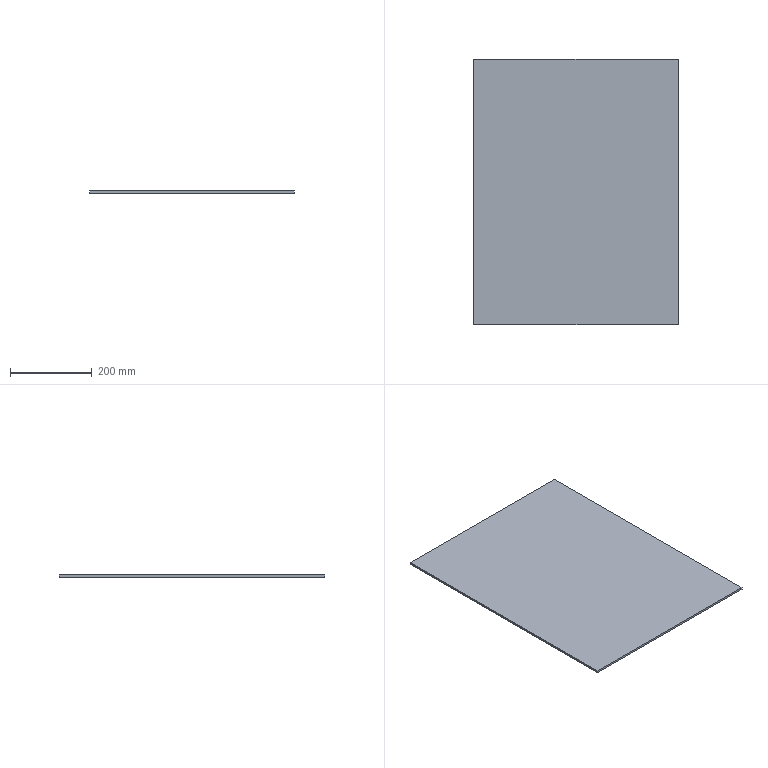Component | SolidWorks | BrownAcrylicPlate-5_BrownAcrylicPlate-5-1 | 1 solid | 6 faces | box 500 x 650 x 5 mm | volume 1625000 mm3 | plane 6
build123d program:
from build123d import *

# Parameters (mm, degrees)
SKETCH1_W           = 500
SKETCH1_H           = 650
BOSS_EXTRUDE1_DEPTH = 5


with BuildPart() as part:
    # Sketch1 → Boss-Extrude1 (new body)
    with BuildSketch(Plane(origin=(0, 0, 0), x_dir=(1, 0, 0), z_dir=(0, 1, 0))):
        Rectangle(SKETCH1_W, SKETCH1_H)
    extrude(amount=BOSS_EXTRUDE1_DEPTH)


solid = part.part

# Placed as in the assembly
solid = solid.moved(Location((335.689, 1675.552, -2328.5), (90, 0, 0)))
STEP:
#1=COLOUR_RGB('',0.7922,0.8196,0.9333);
#2=FILL_AREA_STYLE_COLOUR('',#1);
#3=FILL_AREA_STYLE('',(#2));
#4=SURFACE_STYLE_FILL_AREA(#3);
#5=SURFACE_SIDE_STYLE('',(#4));
#6=SURFACE_STYLE_USAGE(.BOTH.,#5);
#7=PRESENTATION_STYLE_ASSIGNMENT((#6));
#8=CARTESIAN_POINT('',(23.059,53.171,-91.673));
#9=VERTEX_POINT('',#8);
#10=CARTESIAN_POINT('',(23.059,78.762,-91.673));
#11=VERTEX_POINT('',#10);
#12=CARTESIAN_POINT('',(23.059,78.762,-91.673));
#13=DIRECTION('',(0.,1.,-0.));
#14=VECTOR('',#13,39.37);
#15=LINE('',#12,#14);
#16=EDGE_CURVE('',#9,#11,#15,.T.);
#17=ORIENTED_EDGE('',*,*,#16,.T.);
#18=CARTESIAN_POINT('',(23.059,78.762,-91.476));
#19=VERTEX_POINT('',#18);
#20=CARTESIAN_POINT('',(23.059,78.762,-91.476));
#21=DIRECTION('',(-0.,-0.,-1.));
#22=VECTOR('',#21,39.37);
#23=LINE('',#20,#22);
#24=EDGE_CURVE('',#19,#11,#23,.T.);
#25=ORIENTED_EDGE('',*,*,#24,.F.);
#26=CARTESIAN_POINT('',(23.059,53.171,-91.476));
#27=VERTEX_POINT('',#26);
#28=CARTESIAN_POINT('',(23.059,78.762,-91.476));
#29=DIRECTION('',(0.,1.,-0.));
#30=VECTOR('',#29,39.37);
#31=LINE('',#28,#30);
#32=EDGE_CURVE('',#27,#19,#31,.T.);
#33=ORIENTED_EDGE('',*,*,#32,.F.);
#34=CARTESIAN_POINT('',(23.059,53.171,-91.476));
#35=DIRECTION('',(-0.,-0.,-1.));
#36=VECTOR('',#35,39.37);
#37=LINE('',#34,#36);
#38=EDGE_CURVE('',#27,#9,#37,.T.);
#39=ORIENTED_EDGE('',*,*,#38,.T.);
#40=EDGE_LOOP('',(#17,#25,#33,#39));
#41=FACE_OUTER_BOUND('',#40,.T.);
#42=CARTESIAN_POINT('',(23.059,78.762,-91.476));
#43=DIRECTION('',(-1.,0.,0.));
#44=DIRECTION('',(-0.,-1.,0.));
#45=AXIS2_PLACEMENT_3D('',#42,#43,#44);
#46=PLANE('',#45);
#47=ADVANCED_FACE('',(#41),#46,.F.);
#48=CARTESIAN_POINT('',(3.374,78.762,-91.673));
#49=VERTEX_POINT('',#48);
#50=CARTESIAN_POINT('',(3.374,78.762,-91.673));
#51=DIRECTION('',(-1.,0.,0.));
#52=VECTOR('',#51,39.37);
#53=LINE('',#50,#52);
#54=EDGE_CURVE('',#11,#49,#53,.T.);
#55=ORIENTED_EDGE('',*,*,#54,.T.);
#56=CARTESIAN_POINT('',(3.374,78.762,-91.476));
#57=VERTEX_POINT('',#56);
#58=CARTESIAN_POINT('',(3.374,78.762,-91.476));
#59=DIRECTION('',(-0.,-0.,-1.));
#60=VECTOR('',#59,39.37);
#61=LINE('',#58,#60);
#62=EDGE_CURVE('',#57,#49,#61,.T.);
#63=ORIENTED_EDGE('',*,*,#62,.F.);
#64=CARTESIAN_POINT('',(3.374,78.762,-91.476));
#65=DIRECTION('',(-1.,0.,0.));
#66=VECTOR('',#65,39.37);
#67=LINE('',#64,#66);
#68=EDGE_CURVE('',#19,#57,#67,.T.);
#69=ORIENTED_EDGE('',*,*,#68,.F.);
#70=ORIENTED_EDGE('',*,*,#24,.T.);
#71=EDGE_LOOP('',(#55,#63,#69,#70));
#72=FACE_OUTER_BOUND('',#71,.T.);
#73=CARTESIAN_POINT('',(3.374,78.762,-91.476));
#74=DIRECTION('',(-0.,-1.,0.));
#75=DIRECTION('',(1.,-0.,-0.));
#76=AXIS2_PLACEMENT_3D('',#73,#74,#75);
#77=PLANE('',#76);
#78=ADVANCED_FACE('',(#72),#77,.F.);
#79=CARTESIAN_POINT('',(3.374,53.171,-91.673));
#80=VERTEX_POINT('',#79);
#81=CARTESIAN_POINT('',(3.374,78.762,-91.673));
#82=DIRECTION('',(-0.,-1.,0.));
#83=VECTOR('',#82,39.37);
#84=LINE('',#81,#83);
#85=EDGE_CURVE('',#49,#80,#84,.T.);
#86=ORIENTED_EDGE('',*,*,#85,.T.);
#87=CARTESIAN_POINT('',(3.374,53.171,-91.476));
#88=VERTEX_POINT('',#87);
#89=CARTESIAN_POINT('',(3.374,53.171,-91.476));
#90=DIRECTION('',(-0.,-0.,-1.));
#91=VECTOR('',#90,39.37);
#92=LINE('',#89,#91);
#93=EDGE_CURVE('',#88,#80,#92,.T.);
#94=ORIENTED_EDGE('',*,*,#93,.F.);
#95=CARTESIAN_POINT('',(3.374,78.762,-91.476));
#96=DIRECTION('',(-0.,-1.,0.));
#97=VECTOR('',#96,39.37);
#98=LINE('',#95,#97);
#99=EDGE_CURVE('',#57,#88,#98,.T.);
#100=ORIENTED_EDGE('',*,*,#99,.F.);
#101=ORIENTED_EDGE('',*,*,#62,.T.);
#102=EDGE_LOOP('',(#86,#94,#100,#101));
#103=FACE_OUTER_BOUND('',#102,.T.);
#104=CARTESIAN_POINT('',(3.374,78.762,-91.476));
#105=DIRECTION('',(1.,-0.,-0.));
#106=DIRECTION('',(0.,1.,-0.));
#107=AXIS2_PLACEMENT_3D('',#104,#105,#106);
#108=PLANE('',#107);
#109=ADVANCED_FACE('',(#103),#108,.F.);
#110=CARTESIAN_POINT('',(3.374,53.171,-91.673));
#111=DIRECTION('',(1.,-0.,-0.));
#112=VECTOR('',#111,39.37);
#113=LINE('',#110,#112);
#114=EDGE_CURVE('',#80,#9,#113,.T.);
#115=ORIENTED_EDGE('',*,*,#114,.T.);
#116=ORIENTED_EDGE('',*,*,#38,.F.);
#117=CARTESIAN_POINT('',(3.374,53.171,-91.476));
#118=DIRECTION('',(1.,-0.,-0.));
#119=VECTOR('',#118,39.37);
#120=LINE('',#117,#119);
#121=EDGE_CURVE('',#88,#27,#120,.T.);
#122=ORIENTED_EDGE('',*,*,#121,.F.);
#123=ORIENTED_EDGE('',*,*,#93,.T.);
#124=EDGE_LOOP('',(#115,#116,#122,#123));
#125=FACE_OUTER_BOUND('',#124,.T.);
#126=CARTESIAN_POINT('',(3.374,53.171,-91.476));
#127=DIRECTION('',(0.,1.,-0.));
#128=DIRECTION('',(-1.,0.,0.));
#129=AXIS2_PLACEMENT_3D('',#126,#127,#128);
#130=PLANE('',#129);
#131=ADVANCED_FACE('',(#125),#130,.F.);
#132=ORIENTED_EDGE('',*,*,#32,.T.);
#133=ORIENTED_EDGE('',*,*,#68,.T.);
#134=ORIENTED_EDGE('',*,*,#99,.T.);
#135=ORIENTED_EDGE('',*,*,#121,.T.);
#136=EDGE_LOOP('',(#132,#133,#134,#135));
#137=FACE_OUTER_BOUND('',#136,.T.);
#138=CARTESIAN_POINT('',(13.216,65.967,-91.476));
#139=DIRECTION('',(0.,0.,1.));
#140=DIRECTION('',(-0.,-1.,0.));
#141=AXIS2_PLACEMENT_3D('',#138,#139,#140);
#142=PLANE('',#141);
#143=ADVANCED_FACE('',(#137),#142,.T.);
#144=ORIENTED_EDGE('',*,*,#16,.F.);
#145=ORIENTED_EDGE('',*,*,#114,.F.);
#146=ORIENTED_EDGE('',*,*,#85,.F.);
#147=ORIENTED_EDGE('',*,*,#54,.F.);
#148=EDGE_LOOP('',(#144,#145,#146,#147));
#149=FACE_OUTER_BOUND('',#148,.T.);
#150=CARTESIAN_POINT('',(13.216,65.967,-91.673));
#151=DIRECTION('',(0.,0.,1.));
#152=DIRECTION('',(-0.,-1.,0.));
#153=AXIS2_PLACEMENT_3D('',#150,#151,#152);
#154=PLANE('',#153);
#155=ADVANCED_FACE('',(#149),#154,.F.);
#156=CLOSED_SHELL('',(#47,#78,#109,#131,#143,#155));
#157=MANIFOLD_SOLID_BREP('',#156);
#158=STYLED_ITEM('',(#7),#157);
#159=PRESENTATION_LAYER_ASSIGNMENT('','',(#158));
#160=(LENGTH_UNIT()NAMED_UNIT(*)SI_UNIT($,.METRE.));
#161=LENGTH_MEASURE_WITH_UNIT(LENGTH_MEASURE(0.0254),#160);
#162=DIMENSIONAL_EXPONENTS(1.,0.,0.,0.,0.,0.,0.);
#163=(CONVERSION_BASED_UNIT('',#161)LENGTH_UNIT()NAMED_UNIT(#162));
#164=UNCERTAINTY_MEASURE_WITH_UNIT(LENGTH_MEASURE(0.00001),#163,'','');
#165=(NAMED_UNIT(*)PLANE_ANGLE_UNIT()SI_UNIT($,.RADIAN.));
#166=(NAMED_UNIT(*)SI_UNIT($,.STERADIAN.)SOLID_ANGLE_UNIT());
#167=(GEOMETRIC_REPRESENTATION_CONTEXT(3)GLOBAL_UNCERTAINTY_ASSIGNED_CONTEXT((#164))GLOBAL_UNIT_ASSIGNED_CONTEXT((#163,#165,#166))REPRESENTATION_CONTEXT('',''));
#168=MECHANICAL_DESIGN_GEOMETRIC_PRESENTATION_REPRESENTATION('',(#158),#167);
#169=CARTESIAN_POINT('',(0.,0.,0.));
#170=DIRECTION('',(0.,0.,1.));
#171=DIRECTION('',(1.,0.,0.));
#172=AXIS2_PLACEMENT_3D('',#169,#170,#171);
#173=(LENGTH_UNIT()NAMED_UNIT(*)SI_UNIT($,.METRE.));
#174=LENGTH_MEASURE_WITH_UNIT(LENGTH_MEASURE(0.0254),#173);
#175=DIMENSIONAL_EXPONENTS(1.,0.,0.,0.,0.,0.,0.);
#176=(CONVERSION_BASED_UNIT('',#174)LENGTH_UNIT()NAMED_UNIT(#175));
#177=UNCERTAINTY_MEASURE_WITH_UNIT(LENGTH_MEASURE(0.00001),#176,'','');
#178=(NAMED_UNIT(*)PLANE_ANGLE_UNIT()SI_UNIT($,.RADIAN.));
#179=(NAMED_UNIT(*)SI_UNIT($,.STERADIAN.)SOLID_ANGLE_UNIT());
#180=(GEOMETRIC_REPRESENTATION_CONTEXT(3)GLOBAL_UNCERTAINTY_ASSIGNED_CONTEXT((#177))GLOBAL_UNIT_ASSIGNED_CONTEXT((#176,#178,#179))REPRESENTATION_CONTEXT('',''));
#181=ADVANCED_BREP_SHAPE_REPRESENTATION('',(#157,#172),#180);